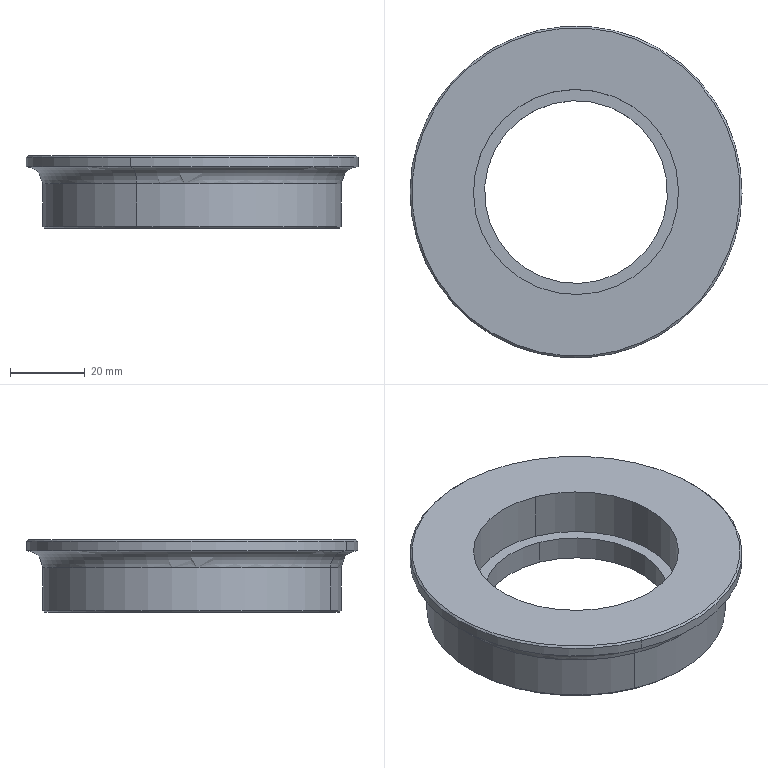Component | SolidWorks | 12AOuterSideWheel-EngravingAndMillingAxis-1_12AOuterSideWheel-3 | 1 solid | 17 faces | box 89 x 89 x 19.5 mm | volume 59512 mm3 | cylinder 8 | cone 4 | plane 3 | torus 2 | commonest cylinder face diameters 55 x2 89 x2 80 x2 49 x2 | material Cr12MoV
build123d program:
from build123d import *

# Parameters (mm, degrees)
CHAMFER1_SIZE = 0.5


with BuildPart() as part:
    # Sketch1 → Revolve1 (revolve)
    with BuildSketch(Plane.XY, mode=Mode.PRIVATE) as revolve1_sk:
        with BuildLine():
            Line((0.5, 44.5), (3, 44.5))
            ThreePointArc((3, 44.5), (4.318, 41.318), (7.5, 40))
            Line((7.5, 40), (19.5, 40))
            Line((19.5, 40), (19.5, 24.5))
            Line((19.5, 24.5), (13, 24.5))
            Line((13, 24.5), (13, 27.5))
            Line((13, 27.5), (0, 27.5))
            Line((0, 27.5), (0, 44))
            Line((0, 44), (0.5, 44.5))
        make_face()
    revolve(revolve1_sk.sketch.rotate(Axis((0, 0, 0), (1, 0, 0)), 90), axis=Axis((0, 0, 0), (1, 0, 0)))

    # Chamfer1
    chamfer1_edges = [part.edges().sort_by_distance(p)[0] for p in [
        (19.5, 0, -40),
    ]]
    chamfer(chamfer1_edges, length=CHAMFER1_SIZE)


solid = part.part

# Placed as in the assembly
solid = solid.moved(Location((271.598, 136.538, 56.25), (0, 90, 0)))
STEP:
#1=CARTESIAN_POINT('',(10.116,3.931,1.447));
#2=VERTEX_POINT('',#1);
#3=CARTESIAN_POINT('',(11.27,6.82,1.447));
#4=VERTEX_POINT('',#3);
#5=CARTESIAN_POINT('',(10.693,5.376,1.447));
#6=DIRECTION('',(-0.,-0.,-1.));
#7=DIRECTION('',(0.3711,0.9286,0.));
#8=AXIS2_PLACEMENT_3D('',#5,#6,#7);
#9=CIRCLE('',#8,1.555);
#10=EDGE_CURVE('',#2,#4,#9,.T.);
#11=ORIENTED_EDGE('',*,*,#10,.F.);
#12=CARTESIAN_POINT('',(10.108,3.913,1.467));
#13=VERTEX_POINT('',#12);
#14=CARTESIAN_POINT('',(10.108,3.913,1.467));
#15=DIRECTION('',(-0.2624,-0.6566,0.7071));
#16=VECTOR('',#15,39.37);
#17=LINE('',#14,#16);
#18=EDGE_CURVE('',#2,#13,#17,.T.);
#19=ORIENTED_EDGE('',*,*,#18,.T.);
#20=CARTESIAN_POINT('',(11.277,6.838,1.467));
#21=VERTEX_POINT('',#20);
#22=CARTESIAN_POINT('',(10.693,5.376,1.467));
#23=DIRECTION('',(0.,0.,1.));
#24=DIRECTION('',(0.3711,0.9286,0.));
#25=AXIS2_PLACEMENT_3D('',#22,#23,#24);
#26=CIRCLE('',#25,1.575);
#27=EDGE_CURVE('',#21,#13,#26,.T.);
#28=ORIENTED_EDGE('',*,*,#27,.F.);
#29=CARTESIAN_POINT('',(11.277,6.838,1.467));
#30=DIRECTION('',(0.2624,0.6566,0.7071));
#31=VECTOR('',#30,39.37);
#32=LINE('',#29,#31);
#33=EDGE_CURVE('',#4,#21,#32,.T.);
#34=ORIENTED_EDGE('',*,*,#33,.F.);
#35=EDGE_LOOP('',(#11,#19,#28,#34));
#36=FACE_OUTER_BOUND('',#35,.T.);
#37=CARTESIAN_POINT('',(10.693,5.376,1.467));
#38=DIRECTION('',(0.,0.,1.));
#39=DIRECTION('',(0.3711,0.9286,0.));
#40=AXIS2_PLACEMENT_3D('',#37,#38,#39);
#41=CONICAL_SURFACE('',#40,1.575,0.7854);
#42=ADVANCED_FACE('',(#36),#41,.T.);
#43=CARTESIAN_POINT('',(10.291,4.37,1.703));
#44=VERTEX_POINT('',#43);
#45=CARTESIAN_POINT('',(11.095,6.381,1.703));
#46=VERTEX_POINT('',#45);
#47=CARTESIAN_POINT('',(10.693,5.376,1.703));
#48=DIRECTION('',(0.,0.,1.));
#49=DIRECTION('',(0.3711,0.9286,0.));
#50=AXIS2_PLACEMENT_3D('',#47,#48,#49);
#51=CIRCLE('',#50,1.083);
#52=EDGE_CURVE('',#44,#46,#51,.T.);
#53=ORIENTED_EDGE('',*,*,#52,.F.);
#54=CARTESIAN_POINT('',(10.291,4.37,2.215));
#55=VERTEX_POINT('',#54);
#56=CARTESIAN_POINT('',(10.291,4.37,2.215));
#57=DIRECTION('',(0.,0.,1.));
#58=VECTOR('',#57,39.37);
#59=LINE('',#56,#58);
#60=EDGE_CURVE('',#44,#55,#59,.T.);
#61=ORIENTED_EDGE('',*,*,#60,.T.);
#62=CARTESIAN_POINT('',(11.095,6.381,2.215));
#63=VERTEX_POINT('',#62);
#64=CARTESIAN_POINT('',(10.693,5.376,2.215));
#65=DIRECTION('',(0.,0.,1.));
#66=DIRECTION('',(0.3711,0.9286,0.));
#67=AXIS2_PLACEMENT_3D('',#64,#65,#66);
#68=CIRCLE('',#67,1.083);
#69=EDGE_CURVE('',#55,#63,#68,.T.);
#70=ORIENTED_EDGE('',*,*,#69,.T.);
#71=CARTESIAN_POINT('',(11.095,6.381,2.215));
#72=DIRECTION('',(0.,0.,1.));
#73=VECTOR('',#72,39.37);
#74=LINE('',#71,#73);
#75=EDGE_CURVE('',#46,#63,#74,.T.);
#76=ORIENTED_EDGE('',*,*,#75,.F.);
#77=EDGE_LOOP('',(#53,#61,#70,#76));
#78=FACE_OUTER_BOUND('',#77,.T.);
#79=CARTESIAN_POINT('',(10.693,5.376,2.215));
#80=DIRECTION('',(0.,0.,1.));
#81=DIRECTION('',(0.3711,0.9286,0.));
#82=AXIS2_PLACEMENT_3D('',#79,#80,#81);
#83=CYLINDRICAL_SURFACE('',#82,1.083);
#84=ADVANCED_FACE('',(#78),#83,.F.);
#85=CARTESIAN_POINT('',(11.336,6.984,2.215));
#86=VERTEX_POINT('',#85);
#87=CARTESIAN_POINT('',(10.05,3.767,2.215));
#88=VERTEX_POINT('',#87);
#89=CARTESIAN_POINT('',(10.693,5.376,2.215));
#90=DIRECTION('',(0.,0.,1.));
#91=DIRECTION('',(0.3711,0.9286,0.));
#92=AXIS2_PLACEMENT_3D('',#89,#90,#91);
#93=CIRCLE('',#92,1.732);
#94=EDGE_CURVE('',#86,#88,#93,.T.);
#95=ORIENTED_EDGE('',*,*,#94,.F.);
#96=CARTESIAN_POINT('',(11.343,7.002,2.195));
#97=VERTEX_POINT('',#96);
#98=CARTESIAN_POINT('',(11.343,7.002,2.195));
#99=DIRECTION('',(0.2624,0.6566,-0.7071));
#100=VECTOR('',#99,39.37);
#101=LINE('',#98,#100);
#102=EDGE_CURVE('',#86,#97,#101,.T.);
#103=ORIENTED_EDGE('',*,*,#102,.T.);
#104=CARTESIAN_POINT('',(10.043,3.749,2.195));
#105=VERTEX_POINT('',#104);
#106=CARTESIAN_POINT('',(10.693,5.376,2.195));
#107=DIRECTION('',(0.,0.,1.));
#108=DIRECTION('',(0.3711,0.9286,0.));
#109=AXIS2_PLACEMENT_3D('',#106,#107,#108);
#110=CIRCLE('',#109,1.752);
#111=EDGE_CURVE('',#97,#105,#110,.T.);
#112=ORIENTED_EDGE('',*,*,#111,.T.);
#113=CARTESIAN_POINT('',(10.043,3.749,2.195));
#114=DIRECTION('',(-0.2624,-0.6566,-0.7071));
#115=VECTOR('',#114,39.37);
#116=LINE('',#113,#115);
#117=EDGE_CURVE('',#88,#105,#116,.T.);
#118=ORIENTED_EDGE('',*,*,#117,.F.);
#119=EDGE_LOOP('',(#95,#103,#112,#118));
#120=FACE_OUTER_BOUND('',#119,.T.);
#121=CARTESIAN_POINT('',(10.693,5.376,2.195));
#122=DIRECTION('',(-0.,-0.,-1.));
#123=DIRECTION('',(-0.3711,-0.9286,0.));
#124=AXIS2_PLACEMENT_3D('',#121,#122,#123);
#125=CONICAL_SURFACE('',#124,1.752,0.7854);
#126=ADVANCED_FACE('',(#120),#125,.T.);
#127=CARTESIAN_POINT('',(11.343,7.002,2.096));
#128=VERTEX_POINT('',#127);
#129=CARTESIAN_POINT('',(10.043,3.749,2.096));
#130=VERTEX_POINT('',#129);
#131=CARTESIAN_POINT('',(10.693,5.376,2.096));
#132=DIRECTION('',(0.,0.,1.));
#133=DIRECTION('',(0.3711,0.9286,0.));
#134=AXIS2_PLACEMENT_3D('',#131,#132,#133);
#135=CIRCLE('',#134,1.752);
#136=EDGE_CURVE('',#128,#130,#135,.T.);
#137=ORIENTED_EDGE('',*,*,#136,.T.);
#138=CARTESIAN_POINT('',(10.043,3.749,2.215));
#139=DIRECTION('',(0.,0.,1.));
#140=VECTOR('',#139,39.37);
#141=LINE('',#138,#140);
#142=EDGE_CURVE('',#130,#105,#141,.T.);
#143=ORIENTED_EDGE('',*,*,#142,.T.);
#144=ORIENTED_EDGE('',*,*,#111,.F.);
#145=CARTESIAN_POINT('',(11.343,7.002,2.215));
#146=DIRECTION('',(0.,0.,1.));
#147=VECTOR('',#146,39.37);
#148=LINE('',#145,#147);
#149=EDGE_CURVE('',#128,#97,#148,.T.);
#150=ORIENTED_EDGE('',*,*,#149,.F.);
#151=EDGE_LOOP('',(#137,#143,#144,#150));
#152=FACE_OUTER_BOUND('',#151,.T.);
#153=CARTESIAN_POINT('',(10.693,5.376,2.215));
#154=DIRECTION('',(0.,0.,1.));
#155=DIRECTION('',(0.3711,0.9286,0.));
#156=AXIS2_PLACEMENT_3D('',#153,#154,#155);
#157=CYLINDRICAL_SURFACE('',#156,1.752);
#158=ADVANCED_FACE('',(#152),#157,.T.);
#159=CARTESIAN_POINT('',(10.693,5.376,2.096));
#160=DIRECTION('',(0.,0.,1.));
#161=DIRECTION('',(0.3711,0.9286,0.));
#162=AXIS2_PLACEMENT_3D('',#159,#160,#161);
#163=CIRCLE('',#162,1.752);
#164=EDGE_CURVE('',#130,#128,#163,.T.);
#165=ORIENTED_EDGE('',*,*,#164,.F.);
#166=CARTESIAN_POINT('',(10.108,3.913,1.919));
#167=VERTEX_POINT('',#166);
#168=CARTESIAN_POINT('',(10.043,3.749,1.919));
#169=DIRECTION('',(-0.9286,0.3711,-0.));
#170=DIRECTION('',(-0.3711,-0.9286,0.));
#171=AXIS2_PLACEMENT_3D('',#168,#169,#170);
#172=CIRCLE('',#171,0.1772);
#173=EDGE_CURVE('',#130,#167,#172,.T.);
#174=ORIENTED_EDGE('',*,*,#173,.T.);
#175=CARTESIAN_POINT('',(11.277,6.838,1.919));
#176=VERTEX_POINT('',#175);
#177=CARTESIAN_POINT('',(10.693,5.376,1.919));
#178=DIRECTION('',(0.,0.,1.));
#179=DIRECTION('',(0.3711,0.9286,0.));
#180=AXIS2_PLACEMENT_3D('',#177,#178,#179);
#181=CIRCLE('',#180,1.575);
#182=EDGE_CURVE('',#167,#176,#181,.T.);
#183=ORIENTED_EDGE('',*,*,#182,.T.);
#184=CARTESIAN_POINT('',(11.343,7.002,1.919));
#185=DIRECTION('',(0.9286,-0.3711,0.));
#186=DIRECTION('',(0.3711,0.9286,0.));
#187=AXIS2_PLACEMENT_3D('',#184,#185,#186);
#188=CIRCLE('',#187,0.1772);
#189=EDGE_CURVE('',#128,#176,#188,.T.);
#190=ORIENTED_EDGE('',*,*,#189,.F.);
#191=EDGE_LOOP('',(#165,#174,#183,#190));
#192=FACE_OUTER_BOUND('',#191,.T.);
#193=CARTESIAN_POINT('',(10.693,5.376,1.919));
#194=DIRECTION('',(0.,0.,1.));
#195=DIRECTION('',(0.3711,0.9286,-0.));
#196=AXIS2_PLACEMENT_3D('',#193,#194,#195);
#197=TOROIDAL_SURFACE('',#196,1.752,0.1772);
#198=ADVANCED_FACE('',(#192),#197,.F.);
#199=ORIENTED_EDGE('',*,*,#27,.T.);
#200=CARTESIAN_POINT('',(10.108,3.913,2.215));
#201=DIRECTION('',(0.,0.,1.));
#202=VECTOR('',#201,39.37);
#203=LINE('',#200,#202);
#204=EDGE_CURVE('',#13,#167,#203,.T.);
#205=ORIENTED_EDGE('',*,*,#204,.T.);
#206=CARTESIAN_POINT('',(10.693,5.376,1.919));
#207=DIRECTION('',(0.,0.,1.));
#208=DIRECTION('',(0.3711,0.9286,0.));
#209=AXIS2_PLACEMENT_3D('',#206,#207,#208);
#210=CIRCLE('',#209,1.575);
#211=EDGE_CURVE('',#176,#167,#210,.T.);
#212=ORIENTED_EDGE('',*,*,#211,.F.);
#213=CARTESIAN_POINT('',(11.277,6.838,2.215));
#214=DIRECTION('',(0.,0.,1.));
#215=VECTOR('',#214,39.37);
#216=LINE('',#213,#215);
#217=EDGE_CURVE('',#21,#176,#216,.T.);
#218=ORIENTED_EDGE('',*,*,#217,.F.);
#219=EDGE_LOOP('',(#199,#205,#212,#218));
#220=FACE_OUTER_BOUND('',#219,.T.);
#221=CARTESIAN_POINT('',(10.693,5.376,2.215));
#222=DIRECTION('',(0.,0.,1.));
#223=DIRECTION('',(0.3711,0.9286,0.));
#224=AXIS2_PLACEMENT_3D('',#221,#222,#223);
#225=CYLINDRICAL_SURFACE('',#224,1.575);
#226=ADVANCED_FACE('',(#220),#225,.T.);
#227=CARTESIAN_POINT('',(10.335,4.48,1.447));
#228=VERTEX_POINT('',#227);
#229=CARTESIAN_POINT('',(11.051,6.271,1.447));
#230=VERTEX_POINT('',#229);
#231=CARTESIAN_POINT('',(10.693,5.376,1.447));
#232=DIRECTION('',(0.,0.,1.));
#233=DIRECTION('',(0.3711,0.9286,0.));
#234=AXIS2_PLACEMENT_3D('',#231,#232,#233);
#235=CIRCLE('',#234,0.9646);
#236=EDGE_CURVE('',#228,#230,#235,.T.);
#237=ORIENTED_EDGE('',*,*,#236,.F.);
#238=CARTESIAN_POINT('',(10.335,4.48,1.703));
#239=VERTEX_POINT('',#238);
#240=CARTESIAN_POINT('',(10.335,4.48,2.215));
#241=DIRECTION('',(0.,0.,1.));
#242=VECTOR('',#241,39.37);
#243=LINE('',#240,#242);
#244=EDGE_CURVE('',#228,#239,#243,.T.);
#245=ORIENTED_EDGE('',*,*,#244,.T.);
#246=CARTESIAN_POINT('',(11.051,6.271,1.703));
#247=VERTEX_POINT('',#246);
#248=CARTESIAN_POINT('',(10.693,5.376,1.703));
#249=DIRECTION('',(0.,0.,1.));
#250=DIRECTION('',(0.3711,0.9286,0.));
#251=AXIS2_PLACEMENT_3D('',#248,#249,#250);
#252=CIRCLE('',#251,0.9646);
#253=EDGE_CURVE('',#239,#247,#252,.T.);
#254=ORIENTED_EDGE('',*,*,#253,.T.);
#255=CARTESIAN_POINT('',(11.051,6.271,2.215));
#256=DIRECTION('',(0.,0.,1.));
#257=VECTOR('',#256,39.37);
#258=LINE('',#255,#257);
#259=EDGE_CURVE('',#230,#247,#258,.T.);
#260=ORIENTED_EDGE('',*,*,#259,.F.);
#261=EDGE_LOOP('',(#237,#245,#254,#260));
#262=FACE_OUTER_BOUND('',#261,.T.);
#263=CARTESIAN_POINT('',(10.693,5.376,2.215));
#264=DIRECTION('',(0.,0.,1.));
#265=DIRECTION('',(0.3711,0.9286,0.));
#266=AXIS2_PLACEMENT_3D('',#263,#264,#265);
#267=CYLINDRICAL_SURFACE('',#266,0.9646);
#268=ADVANCED_FACE('',(#262),#267,.F.);
#269=ORIENTED_EDGE('',*,*,#244,.F.);
#270=CARTESIAN_POINT('',(10.693,5.376,1.447));
#271=DIRECTION('',(0.,0.,1.));
#272=DIRECTION('',(0.3711,0.9286,0.));
#273=AXIS2_PLACEMENT_3D('',#270,#271,#272);
#274=CIRCLE('',#273,0.9646);
#275=EDGE_CURVE('',#230,#228,#274,.T.);
#276=ORIENTED_EDGE('',*,*,#275,.F.);
#277=ORIENTED_EDGE('',*,*,#259,.T.);
#278=CARTESIAN_POINT('',(10.693,5.376,1.703));
#279=DIRECTION('',(0.,0.,1.));
#280=DIRECTION('',(0.3711,0.9286,0.));
#281=AXIS2_PLACEMENT_3D('',#278,#279,#280);
#282=CIRCLE('',#281,0.9646);
#283=EDGE_CURVE('',#247,#239,#282,.T.);
#284=ORIENTED_EDGE('',*,*,#283,.T.);
#285=EDGE_LOOP('',(#269,#276,#277,#284));
#286=FACE_OUTER_BOUND('',#285,.T.);
#287=CARTESIAN_POINT('',(10.693,5.376,2.215));
#288=DIRECTION('',(0.,0.,1.));
#289=DIRECTION('',(0.3711,0.9286,0.));
#290=AXIS2_PLACEMENT_3D('',#287,#288,#289);
#291=CYLINDRICAL_SURFACE('',#290,0.9646);
#292=ADVANCED_FACE('',(#286),#291,.F.);
#293=CARTESIAN_POINT('',(10.693,5.376,1.447));
#294=DIRECTION('',(-0.,-0.,-1.));
#295=DIRECTION('',(0.3711,0.9286,0.));
#296=AXIS2_PLACEMENT_3D('',#293,#294,#295);
#297=CIRCLE('',#296,1.555);
#298=EDGE_CURVE('',#4,#2,#297,.T.);
#299=ORIENTED_EDGE('',*,*,#298,.T.);
#300=ORIENTED_EDGE('',*,*,#10,.T.);
#301=EDGE_LOOP('',(#299,#300));
#302=FACE_OUTER_BOUND('',#301,.T.);
#303=ORIENTED_EDGE('',*,*,#275,.T.);
#304=ORIENTED_EDGE('',*,*,#236,.T.);
#305=EDGE_LOOP('',(#303,#304));
#306=FACE_BOUND('',#305,.T.);
#307=CARTESIAN_POINT('',(9.797,5.733,1.447));
#308=DIRECTION('',(0.,0.,1.));
#309=DIRECTION('',(0.3711,0.9286,-0.));
#310=AXIS2_PLACEMENT_3D('',#307,#308,#309);
#311=PLANE('',#310);
#312=ADVANCED_FACE('',(#302,#306),#311,.F.);
#313=ORIENTED_EDGE('',*,*,#204,.F.);
#314=CARTESIAN_POINT('',(10.693,5.376,1.467));
#315=DIRECTION('',(0.,0.,1.));
#316=DIRECTION('',(0.3711,0.9286,0.));
#317=AXIS2_PLACEMENT_3D('',#314,#315,#316);
#318=CIRCLE('',#317,1.575);
#319=EDGE_CURVE('',#13,#21,#318,.T.);
#320=ORIENTED_EDGE('',*,*,#319,.T.);
#321=ORIENTED_EDGE('',*,*,#217,.T.);
#322=ORIENTED_EDGE('',*,*,#182,.F.);
#323=EDGE_LOOP('',(#313,#320,#321,#322));
#324=FACE_OUTER_BOUND('',#323,.T.);
#325=CARTESIAN_POINT('',(10.693,5.376,2.215));
#326=DIRECTION('',(0.,0.,1.));
#327=DIRECTION('',(0.3711,0.9286,0.));
#328=AXIS2_PLACEMENT_3D('',#325,#326,#327);
#329=CYLINDRICAL_SURFACE('',#328,1.575);
#330=ADVANCED_FACE('',(#324),#329,.T.);
#331=ORIENTED_EDGE('',*,*,#173,.F.);
#332=ORIENTED_EDGE('',*,*,#136,.F.);
#333=ORIENTED_EDGE('',*,*,#189,.T.);
#334=ORIENTED_EDGE('',*,*,#211,.T.);
#335=EDGE_LOOP('',(#331,#332,#333,#334));
#336=FACE_OUTER_BOUND('',#335,.T.);
#337=CARTESIAN_POINT('',(10.693,5.376,1.919));
#338=DIRECTION('',(0.,0.,1.));
#339=DIRECTION('',(0.3711,0.9286,-0.));
#340=AXIS2_PLACEMENT_3D('',#337,#338,#339);
#341=TOROIDAL_SURFACE('',#340,1.752,0.1772);
#342=ADVANCED_FACE('',(#336),#341,.F.);
#343=ORIENTED_EDGE('',*,*,#142,.F.);
#344=ORIENTED_EDGE('',*,*,#164,.T.);
#345=ORIENTED_EDGE('',*,*,#149,.T.);
#346=CARTESIAN_POINT('',(10.693,5.376,2.195));
#347=DIRECTION('',(0.,0.,1.));
#348=DIRECTION('',(0.3711,0.9286,0.));
#349=AXIS2_PLACEMENT_3D('',#346,#347,#348);
#350=CIRCLE('',#349,1.752);
#351=EDGE_CURVE('',#105,#97,#350,.T.);
#352=ORIENTED_EDGE('',*,*,#351,.F.);
#353=EDGE_LOOP('',(#343,#344,#345,#352));
#354=FACE_OUTER_BOUND('',#353,.T.);
#355=CARTESIAN_POINT('',(10.693,5.376,2.215));
#356=DIRECTION('',(0.,0.,1.));
#357=DIRECTION('',(0.3711,0.9286,0.));
#358=AXIS2_PLACEMENT_3D('',#355,#356,#357);
#359=CYLINDRICAL_SURFACE('',#358,1.752);
#360=ADVANCED_FACE('',(#354),#359,.T.);
#361=ORIENTED_EDGE('',*,*,#102,.F.);
#362=CARTESIAN_POINT('',(10.693,5.376,2.215));
#363=DIRECTION('',(0.,0.,1.));
#364=DIRECTION('',(0.3711,0.9286,0.));
#365=AXIS2_PLACEMENT_3D('',#362,#363,#364);
#366=CIRCLE('',#365,1.732);
#367=EDGE_CURVE('',#88,#86,#366,.T.);
#368=ORIENTED_EDGE('',*,*,#367,.F.);
#369=ORIENTED_EDGE('',*,*,#117,.T.);
#370=ORIENTED_EDGE('',*,*,#351,.T.);
#371=EDGE_LOOP('',(#361,#368,#369,#370));
#372=FACE_OUTER_BOUND('',#371,.T.);
#373=CARTESIAN_POINT('',(10.693,5.376,2.195));
#374=DIRECTION('',(-0.,-0.,-1.));
#375=DIRECTION('',(-0.3711,-0.9286,0.));
#376=AXIS2_PLACEMENT_3D('',#373,#374,#375);
#377=CONICAL_SURFACE('',#376,1.752,0.7854);
#378=ADVANCED_FACE('',(#372),#377,.T.);
#379=CARTESIAN_POINT('',(10.693,5.376,2.215));
#380=DIRECTION('',(0.,0.,1.));
#381=DIRECTION('',(0.3711,0.9286,0.));
#382=AXIS2_PLACEMENT_3D('',#379,#380,#381);
#383=CIRCLE('',#382,1.083);
#384=EDGE_CURVE('',#63,#55,#383,.T.);
#385=ORIENTED_EDGE('',*,*,#384,.F.);
#386=ORIENTED_EDGE('',*,*,#69,.F.);
#387=EDGE_LOOP('',(#385,#386));
#388=FACE_BOUND('',#387,.T.);
#389=ORIENTED_EDGE('',*,*,#367,.T.);
#390=ORIENTED_EDGE('',*,*,#94,.T.);
#391=EDGE_LOOP('',(#389,#390));
#392=FACE_OUTER_BOUND('',#391,.T.);
#393=CARTESIAN_POINT('',(9.687,5.777,2.215));
#394=DIRECTION('',(-0.,-0.,-1.));
#395=DIRECTION('',(-0.3711,-0.9286,0.));
#396=AXIS2_PLACEMENT_3D('',#393,#394,#395);
#397=PLANE('',#396);
#398=ADVANCED_FACE('',(#388,#392),#397,.F.);
#399=ORIENTED_EDGE('',*,*,#60,.F.);
#400=CARTESIAN_POINT('',(10.693,5.376,1.703));
#401=DIRECTION('',(0.,0.,1.));
#402=DIRECTION('',(0.3711,0.9286,0.));
#403=AXIS2_PLACEMENT_3D('',#400,#401,#402);
#404=CIRCLE('',#403,1.083);
#405=EDGE_CURVE('',#46,#44,#404,.T.);
#406=ORIENTED_EDGE('',*,*,#405,.F.);
#407=ORIENTED_EDGE('',*,*,#75,.T.);
#408=ORIENTED_EDGE('',*,*,#384,.T.);
#409=EDGE_LOOP('',(#399,#406,#407,#408));
#410=FACE_OUTER_BOUND('',#409,.T.);
#411=CARTESIAN_POINT('',(10.693,5.376,2.215));
#412=DIRECTION('',(0.,0.,1.));
#413=DIRECTION('',(0.3711,0.9286,0.));
#414=AXIS2_PLACEMENT_3D('',#411,#412,#413);
#415=CYLINDRICAL_SURFACE('',#414,1.083);
#416=ADVANCED_FACE('',(#410),#415,.F.);
#417=ORIENTED_EDGE('',*,*,#283,.F.);
#418=ORIENTED_EDGE('',*,*,#253,.F.);
#419=EDGE_LOOP('',(#417,#418));
#420=FACE_BOUND('',#419,.T.);
#421=ORIENTED_EDGE('',*,*,#405,.T.);
#422=ORIENTED_EDGE('',*,*,#52,.T.);
#423=EDGE_LOOP('',(#421,#422));
#424=FACE_OUTER_BOUND('',#423,.T.);
#425=CARTESIAN_POINT('',(9.687,5.777,1.703));
#426=DIRECTION('',(-0.,-0.,-1.));
#427=DIRECTION('',(-0.3711,-0.9286,0.));
#428=AXIS2_PLACEMENT_3D('',#425,#426,#427);
#429=PLANE('',#428);
#430=ADVANCED_FACE('',(#420,#424),#429,.F.);
#431=ORIENTED_EDGE('',*,*,#18,.F.);
#432=ORIENTED_EDGE('',*,*,#298,.F.);
#433=ORIENTED_EDGE('',*,*,#33,.T.);
#434=ORIENTED_EDGE('',*,*,#319,.F.);
#435=EDGE_LOOP('',(#431,#432,#433,#434));
#436=FACE_OUTER_BOUND('',#435,.T.);
#437=CARTESIAN_POINT('',(10.693,5.376,1.467));
#438=DIRECTION('',(0.,0.,1.));
#439=DIRECTION('',(0.3711,0.9286,0.));
#440=AXIS2_PLACEMENT_3D('',#437,#438,#439);
#441=CONICAL_SURFACE('',#440,1.575,0.7854);
#442=ADVANCED_FACE('',(#436),#441,.T.);
#443=CLOSED_SHELL('',(#42,#84,#126,#158,#198,#226,#268,#292,#312,#330,#342,#360,#378,#398,#416,#430,#442));
#444=MANIFOLD_SOLID_BREP('',#443);
#445=CARTESIAN_POINT('',(0.,0.,0.));
#446=DIRECTION('',(0.,0.,1.));
#447=DIRECTION('',(1.,0.,0.));
#448=AXIS2_PLACEMENT_3D('',#445,#446,#447);
#449=(LENGTH_UNIT()NAMED_UNIT(*)SI_UNIT($,.METRE.));
#450=LENGTH_MEASURE_WITH_UNIT(LENGTH_MEASURE(0.0254),#449);
#451=DIMENSIONAL_EXPONENTS(1.,0.,0.,0.,0.,0.,0.);
#452=(CONVERSION_BASED_UNIT('',#450)LENGTH_UNIT()NAMED_UNIT(#451));
#453=UNCERTAINTY_MEASURE_WITH_UNIT(LENGTH_MEASURE(0.00001),#452,'','');
#454=(NAMED_UNIT(*)PLANE_ANGLE_UNIT()SI_UNIT($,.RADIAN.));
#455=(NAMED_UNIT(*)SI_UNIT($,.STERADIAN.)SOLID_ANGLE_UNIT());
#456=(GEOMETRIC_REPRESENTATION_CONTEXT(3)GLOBAL_UNCERTAINTY_ASSIGNED_CONTEXT((#453))GLOBAL_UNIT_ASSIGNED_CONTEXT((#452,#454,#455))REPRESENTATION_CONTEXT('',''));
#457=ADVANCED_BREP_SHAPE_REPRESENTATION('',(#444,#448),#456);
#458=COLOUR_RGB('',0.7922,0.8196,0.9333);
#459=FILL_AREA_STYLE_COLOUR('',#458);
#460=FILL_AREA_STYLE('',(#459));
#461=SURFACE_STYLE_FILL_AREA(#460);
#462=SURFACE_SIDE_STYLE('',(#461));
#463=SURFACE_STYLE_USAGE(.BOTH.,#462);
#464=PRESENTATION_STYLE_ASSIGNMENT((#463));
#465=STYLED_ITEM('',(#464),#444);
#466=(LENGTH_UNIT()NAMED_UNIT(*)SI_UNIT($,.METRE.));
#467=LENGTH_MEASURE_WITH_UNIT(LENGTH_MEASURE(0.0254),#466);
#468=DIMENSIONAL_EXPONENTS(1.,0.,0.,0.,0.,0.,0.);
#469=(CONVERSION_BASED_UNIT('',#467)LENGTH_UNIT()NAMED_UNIT(#468));
#470=UNCERTAINTY_MEASURE_WITH_UNIT(LENGTH_MEASURE(0.00001),#469,'','');
#471=(NAMED_UNIT(*)PLANE_ANGLE_UNIT()SI_UNIT($,.RADIAN.));
#472=(NAMED_UNIT(*)SI_UNIT($,.STERADIAN.)SOLID_ANGLE_UNIT());
#473=(GEOMETRIC_REPRESENTATION_CONTEXT(3)GLOBAL_UNCERTAINTY_ASSIGNED_CONTEXT((#470))GLOBAL_UNIT_ASSIGNED_CONTEXT((#469,#471,#472))REPRESENTATION_CONTEXT('',''));
#474=MECHANICAL_DESIGN_GEOMETRIC_PRESENTATION_REPRESENTATION('',(#465),#473);
#475=PRESENTATION_LAYER_ASSIGNMENT('','',(#465));